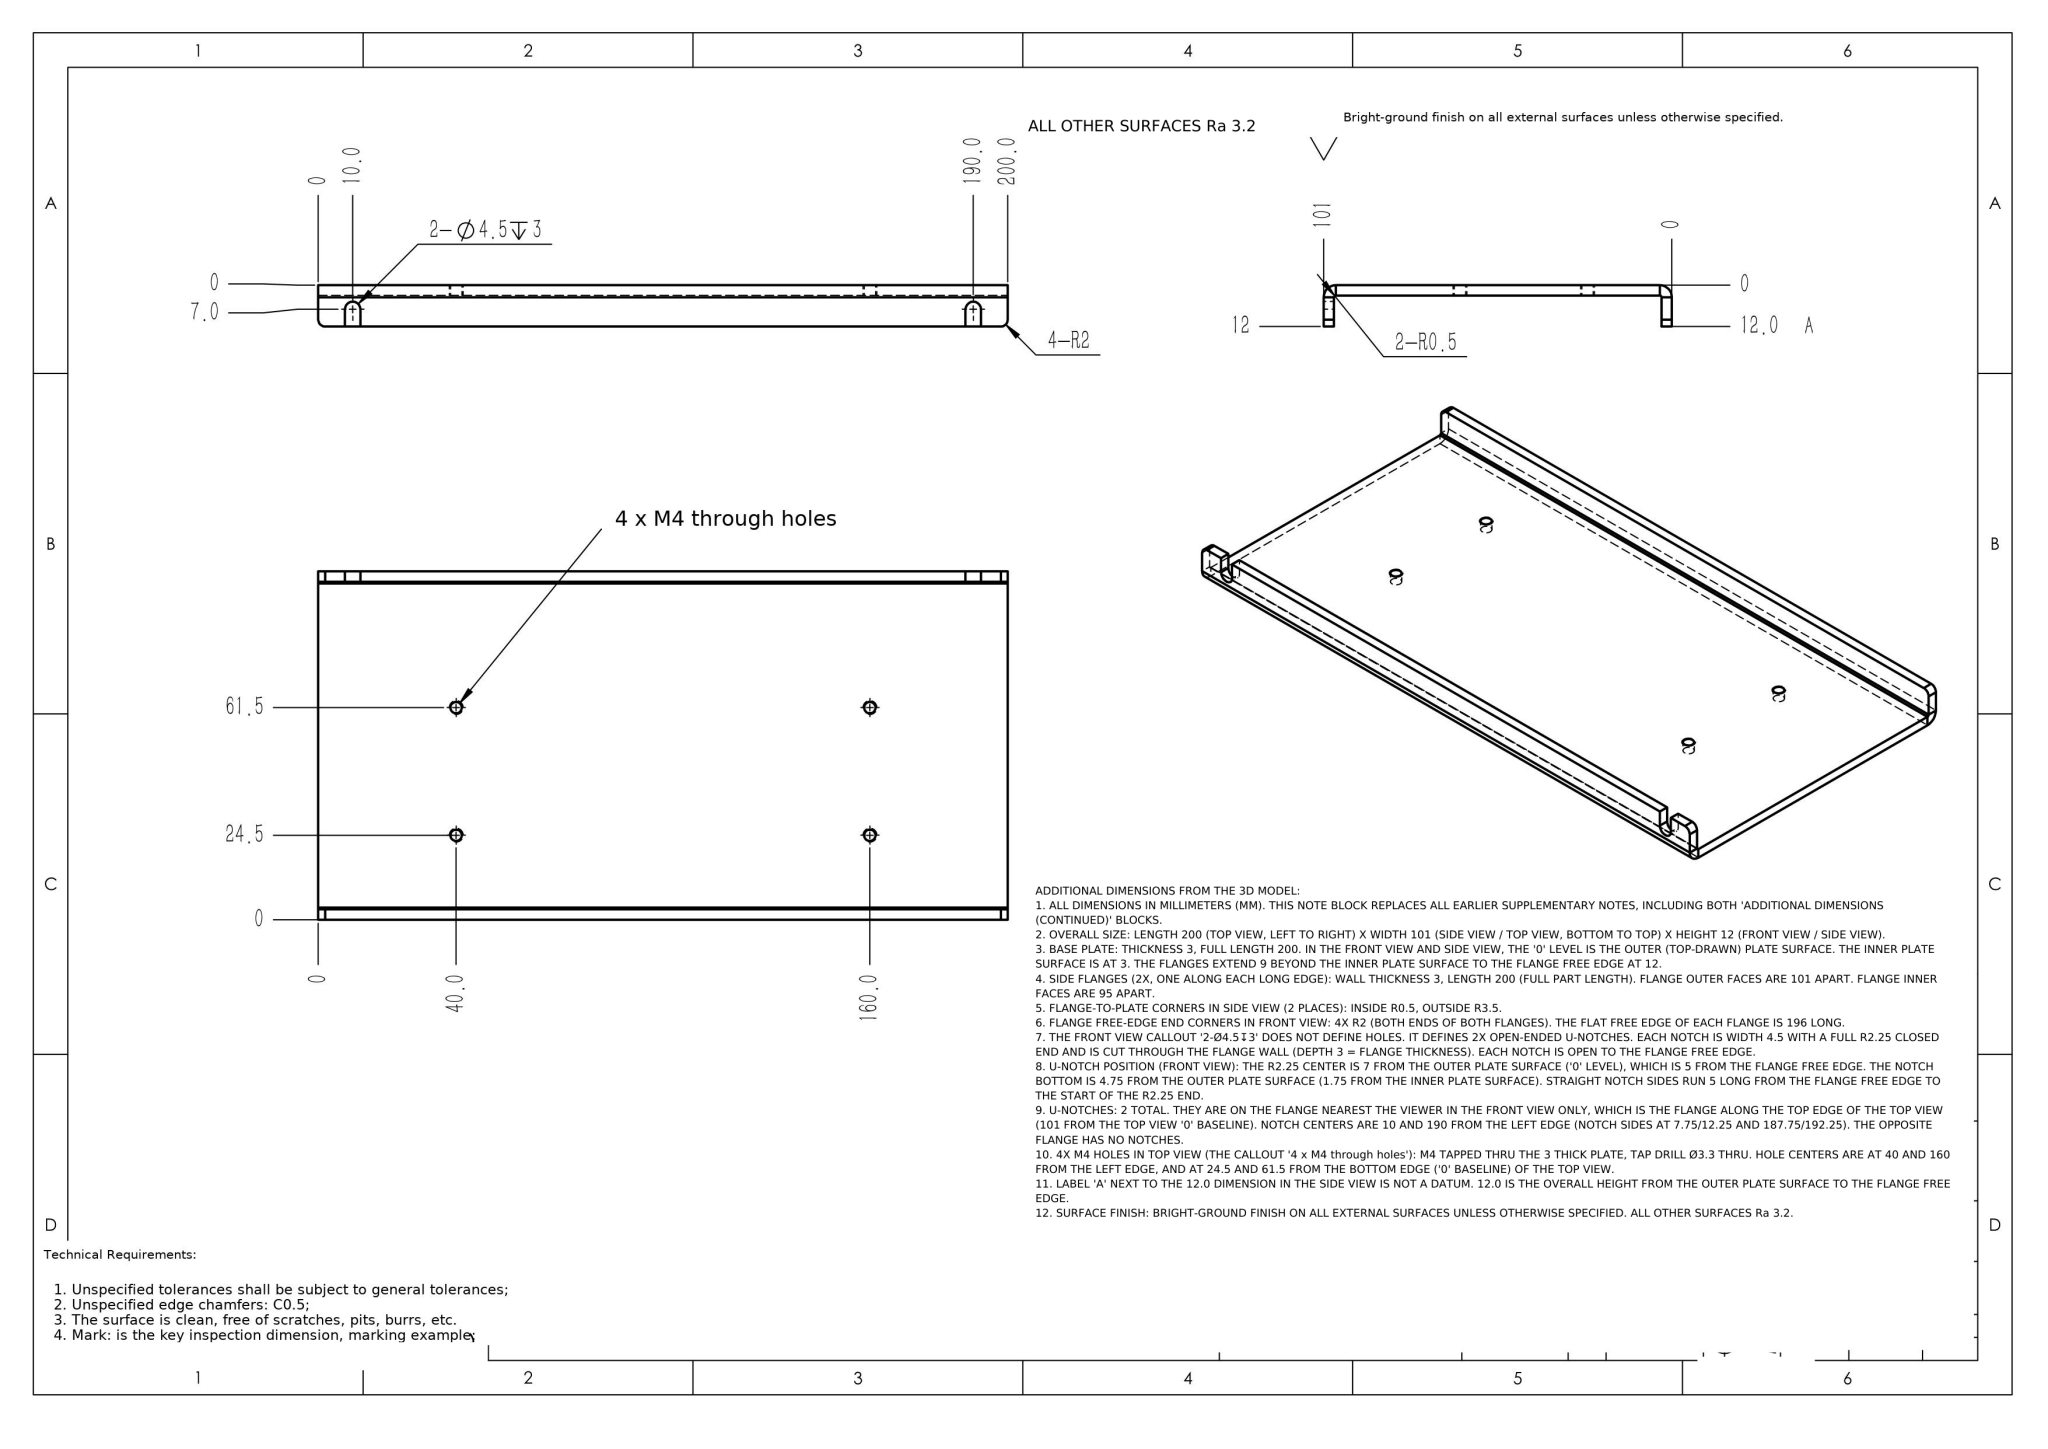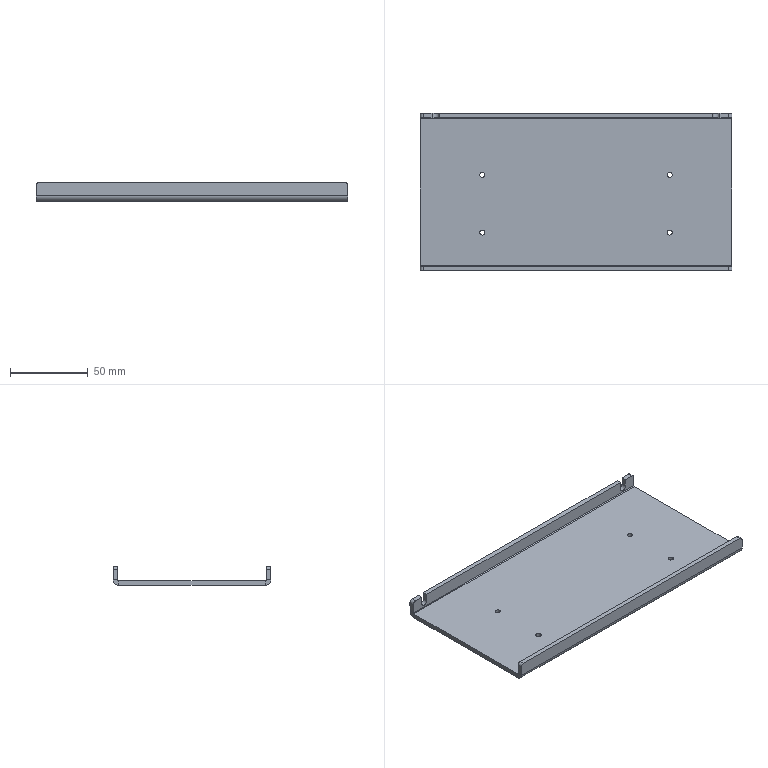Part | NX | mm | 1 solid | 42 faces | box 200 x 101 x 12 mm | volume 70074 mm3 | plane 24 | cylinder 18 | commonest cylinder face diameters 3.3 x8 4 x4 4.5 x2 7 x2 1 x2